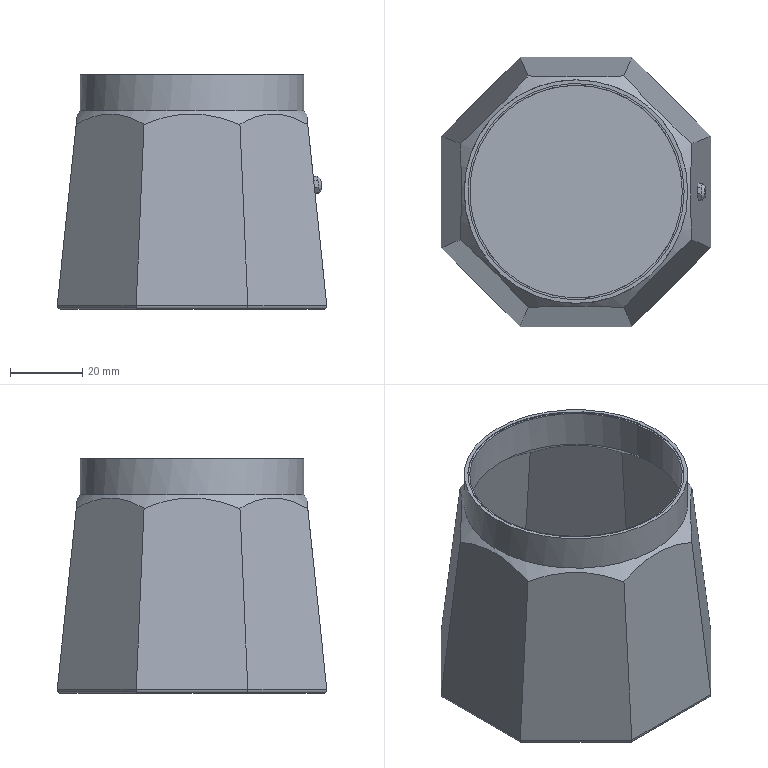Component | NX | MODEL23 | 1 solid | 44 faces | volume 27977 mm3 | plane 29 | cylinder 12 | cone 3 | commonest cylinder face diameters 2 x8 62 x1 60 x1 59 x1 1.5 x1